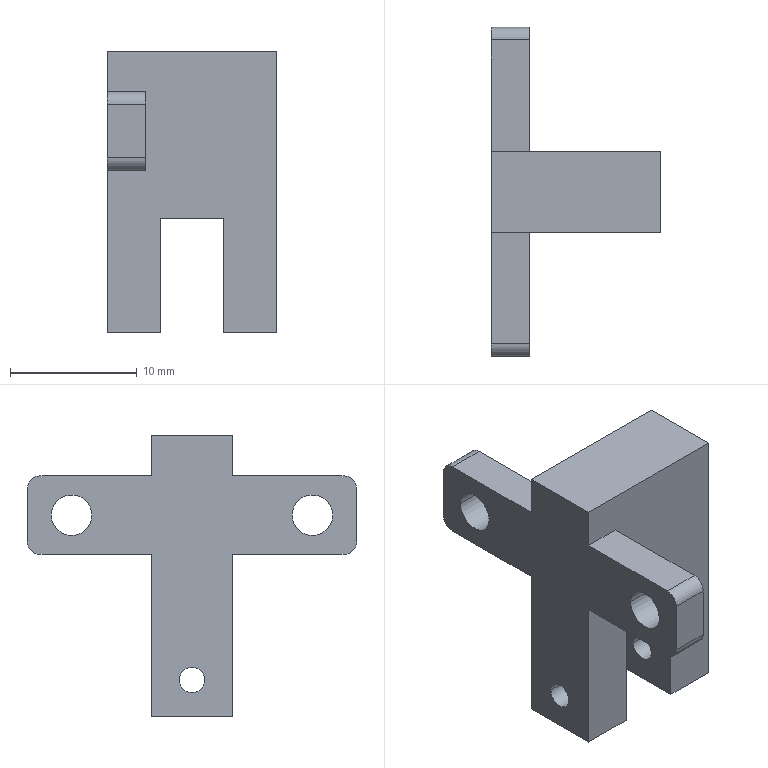Component | SolidWorks | V1ZHXTRR60SecondarySB1-1_v1ZHXTEE-SX672SB1-1 | 1 solid | 30 faces | box 13.4 x 26 x 22.2 mm | volume 1903 mm3 | plane 18 | cylinder 12 | commonest cylinder face diameters 2 x8 3.2 x4
STEP:
#1=COLOUR_RGB('',0.7922,0.8196,0.9333);
#2=FILL_AREA_STYLE_COLOUR('',#1);
#3=FILL_AREA_STYLE('',(#2));
#4=SURFACE_STYLE_FILL_AREA(#3);
#5=SURFACE_SIDE_STYLE('',(#4));
#6=SURFACE_STYLE_USAGE(.BOTH.,#5);
#7=PRESENTATION_STYLE_ASSIGNMENT((#6));
#8=CARTESIAN_POINT('',(9.509,-8.474,18.97));
#9=VERTEX_POINT('',#8);
#10=CARTESIAN_POINT('',(9.509,-8.348,18.97));
#11=VERTEX_POINT('',#10);
#12=CARTESIAN_POINT('',(9.509,-8.411,18.97));
#13=DIRECTION('',(-1.,-0.,-0.));
#14=DIRECTION('',(0.,-1.,-0.));
#15=AXIS2_PLACEMENT_3D('',#12,#13,#14);
#16=CIRCLE('',#15,0.06299);
#17=EDGE_CURVE('',#9,#11,#16,.T.);
#18=ORIENTED_EDGE('',*,*,#17,.T.);
#19=CARTESIAN_POINT('',(9.627,-8.348,18.97));
#20=VERTEX_POINT('',#19);
#21=CARTESIAN_POINT('',(9.627,-8.348,18.97));
#22=DIRECTION('',(1.,0.,0.));
#23=VECTOR('',#22,39.37);
#24=LINE('',#21,#23);
#25=EDGE_CURVE('',#11,#20,#24,.T.);
#26=ORIENTED_EDGE('',*,*,#25,.T.);
#27=CARTESIAN_POINT('',(9.627,-8.474,18.97));
#28=VERTEX_POINT('',#27);
#29=CARTESIAN_POINT('',(9.627,-8.411,18.97));
#30=DIRECTION('',(-1.,-0.,-0.));
#31=DIRECTION('',(0.,-1.,-0.));
#32=AXIS2_PLACEMENT_3D('',#29,#30,#31);
#33=CIRCLE('',#32,0.06299);
#34=EDGE_CURVE('',#28,#20,#33,.T.);
#35=ORIENTED_EDGE('',*,*,#34,.F.);
#36=CARTESIAN_POINT('',(9.627,-8.474,18.97));
#37=DIRECTION('',(1.,0.,0.));
#38=VECTOR('',#37,39.37);
#39=LINE('',#36,#38);
#40=EDGE_CURVE('',#9,#28,#39,.T.);
#41=ORIENTED_EDGE('',*,*,#40,.F.);
#42=EDGE_LOOP('',(#18,#26,#35,#41));
#43=FACE_OUTER_BOUND('',#42,.T.);
#44=CARTESIAN_POINT('',(9.627,-8.411,18.97));
#45=DIRECTION('',(1.,0.,0.));
#46=DIRECTION('',(0.,-1.,-0.));
#47=AXIS2_PLACEMENT_3D('',#44,#45,#46);
#48=CYLINDRICAL_SURFACE('',#47,0.06299);
#49=ADVANCED_FACE('',(#43),#48,.F.);
#50=CARTESIAN_POINT('',(9.509,-7.726,18.97));
#51=VERTEX_POINT('',#50);
#52=CARTESIAN_POINT('',(9.509,-7.6,18.97));
#53=VERTEX_POINT('',#52);
#54=CARTESIAN_POINT('',(9.509,-7.663,18.97));
#55=DIRECTION('',(-1.,-0.,-0.));
#56=DIRECTION('',(0.,-1.,-0.));
#57=AXIS2_PLACEMENT_3D('',#54,#55,#56);
#58=CIRCLE('',#57,0.06299);
#59=EDGE_CURVE('',#51,#53,#58,.T.);
#60=ORIENTED_EDGE('',*,*,#59,.T.);
#61=CARTESIAN_POINT('',(9.627,-7.6,18.97));
#62=VERTEX_POINT('',#61);
#63=CARTESIAN_POINT('',(9.627,-7.6,18.97));
#64=DIRECTION('',(1.,0.,0.));
#65=VECTOR('',#64,39.37);
#66=LINE('',#63,#65);
#67=EDGE_CURVE('',#53,#62,#66,.T.);
#68=ORIENTED_EDGE('',*,*,#67,.T.);
#69=CARTESIAN_POINT('',(9.627,-7.726,18.97));
#70=VERTEX_POINT('',#69);
#71=CARTESIAN_POINT('',(9.627,-7.663,18.97));
#72=DIRECTION('',(-1.,-0.,-0.));
#73=DIRECTION('',(0.,-1.,-0.));
#74=AXIS2_PLACEMENT_3D('',#71,#72,#73);
#75=CIRCLE('',#74,0.06299);
#76=EDGE_CURVE('',#70,#62,#75,.T.);
#77=ORIENTED_EDGE('',*,*,#76,.F.);
#78=CARTESIAN_POINT('',(9.627,-7.726,18.97));
#79=DIRECTION('',(1.,0.,0.));
#80=VECTOR('',#79,39.37);
#81=LINE('',#78,#80);
#82=EDGE_CURVE('',#51,#70,#81,.T.);
#83=ORIENTED_EDGE('',*,*,#82,.F.);
#84=EDGE_LOOP('',(#60,#68,#77,#83));
#85=FACE_OUTER_BOUND('',#84,.T.);
#86=CARTESIAN_POINT('',(9.627,-7.663,18.97));
#87=DIRECTION('',(1.,0.,0.));
#88=DIRECTION('',(0.,-1.,-0.));
#89=AXIS2_PLACEMENT_3D('',#86,#87,#88);
#90=CYLINDRICAL_SURFACE('',#89,0.06299);
#91=ADVANCED_FACE('',(#85),#90,.F.);
#92=CARTESIAN_POINT('',(9.509,-8.076,18.458));
#93=VERTEX_POINT('',#92);
#94=CARTESIAN_POINT('',(9.509,-7.997,18.458));
#95=VERTEX_POINT('',#94);
#96=CARTESIAN_POINT('',(9.509,-8.037,18.458));
#97=DIRECTION('',(-1.,-0.,-0.));
#98=DIRECTION('',(0.,-1.,-0.));
#99=AXIS2_PLACEMENT_3D('',#96,#97,#98);
#100=CIRCLE('',#99,0.03937);
#101=EDGE_CURVE('',#93,#95,#100,.T.);
#102=ORIENTED_EDGE('',*,*,#101,.T.);
#103=CARTESIAN_POINT('',(9.674,-7.997,18.458));
#104=VERTEX_POINT('',#103);
#105=CARTESIAN_POINT('',(10.036,-7.997,18.458));
#106=DIRECTION('',(1.,0.,0.));
#107=VECTOR('',#106,39.37);
#108=LINE('',#105,#107);
#109=EDGE_CURVE('',#95,#104,#108,.T.);
#110=ORIENTED_EDGE('',*,*,#109,.T.);
#111=CARTESIAN_POINT('',(9.674,-8.076,18.458));
#112=VERTEX_POINT('',#111);
#113=CARTESIAN_POINT('',(9.674,-8.037,18.458));
#114=DIRECTION('',(-1.,-0.,-0.));
#115=DIRECTION('',(0.,-1.,-0.));
#116=AXIS2_PLACEMENT_3D('',#113,#114,#115);
#117=CIRCLE('',#116,0.03937);
#118=EDGE_CURVE('',#112,#104,#117,.T.);
#119=ORIENTED_EDGE('',*,*,#118,.F.);
#120=CARTESIAN_POINT('',(10.036,-8.076,18.458));
#121=DIRECTION('',(1.,0.,0.));
#122=VECTOR('',#121,39.37);
#123=LINE('',#120,#122);
#124=EDGE_CURVE('',#93,#112,#123,.T.);
#125=ORIENTED_EDGE('',*,*,#124,.F.);
#126=EDGE_LOOP('',(#102,#110,#119,#125));
#127=FACE_OUTER_BOUND('',#126,.T.);
#128=CARTESIAN_POINT('',(10.036,-8.037,18.458));
#129=DIRECTION('',(1.,0.,0.));
#130=DIRECTION('',(0.,-1.,-0.));
#131=AXIS2_PLACEMENT_3D('',#128,#129,#130);
#132=CYLINDRICAL_SURFACE('',#131,0.03937);
#133=ADVANCED_FACE('',(#127),#132,.F.);
#134=CARTESIAN_POINT('',(9.871,-8.076,18.458));
#135=VERTEX_POINT('',#134);
#136=CARTESIAN_POINT('',(9.871,-7.997,18.458));
#137=VERTEX_POINT('',#136);
#138=CARTESIAN_POINT('',(9.871,-8.037,18.458));
#139=DIRECTION('',(-1.,-0.,-0.));
#140=DIRECTION('',(0.,-1.,-0.));
#141=AXIS2_PLACEMENT_3D('',#138,#139,#140);
#142=CIRCLE('',#141,0.03937);
#143=EDGE_CURVE('',#135,#137,#142,.T.);
#144=ORIENTED_EDGE('',*,*,#143,.T.);
#145=CARTESIAN_POINT('',(10.036,-7.997,18.458));
#146=VERTEX_POINT('',#145);
#147=CARTESIAN_POINT('',(10.036,-7.997,18.458));
#148=DIRECTION('',(1.,0.,0.));
#149=VECTOR('',#148,39.37);
#150=LINE('',#147,#149);
#151=EDGE_CURVE('',#137,#146,#150,.T.);
#152=ORIENTED_EDGE('',*,*,#151,.T.);
#153=CARTESIAN_POINT('',(10.036,-8.076,18.458));
#154=VERTEX_POINT('',#153);
#155=CARTESIAN_POINT('',(10.036,-8.037,18.458));
#156=DIRECTION('',(1.,0.,0.));
#157=DIRECTION('',(0.,-1.,-0.));
#158=AXIS2_PLACEMENT_3D('',#155,#156,#157);
#159=CIRCLE('',#158,0.03937);
#160=EDGE_CURVE('',#146,#154,#159,.T.);
#161=ORIENTED_EDGE('',*,*,#160,.T.);
#162=CARTESIAN_POINT('',(10.036,-8.076,18.458));
#163=DIRECTION('',(1.,0.,0.));
#164=VECTOR('',#163,39.37);
#165=LINE('',#162,#164);
#166=EDGE_CURVE('',#135,#154,#165,.T.);
#167=ORIENTED_EDGE('',*,*,#166,.F.);
#168=EDGE_LOOP('',(#144,#152,#161,#167));
#169=FACE_OUTER_BOUND('',#168,.T.);
#170=CARTESIAN_POINT('',(10.036,-8.037,18.458));
#171=DIRECTION('',(1.,0.,0.));
#172=DIRECTION('',(0.,-1.,-0.));
#173=AXIS2_PLACEMENT_3D('',#170,#171,#172);
#174=CYLINDRICAL_SURFACE('',#173,0.03937);
#175=ADVANCED_FACE('',(#169),#174,.F.);
#176=CARTESIAN_POINT('',(9.509,-7.525,19.053));
#177=VERTEX_POINT('',#176);
#178=CARTESIAN_POINT('',(9.509,-7.564,19.092));
#179=VERTEX_POINT('',#178);
#180=CARTESIAN_POINT('',(9.509,-7.564,19.053));
#181=DIRECTION('',(1.,0.,0.));
#182=DIRECTION('',(-0.,1.,0.));
#183=AXIS2_PLACEMENT_3D('',#180,#181,#182);
#184=CIRCLE('',#183,0.03937);
#185=EDGE_CURVE('',#177,#179,#184,.T.);
#186=ORIENTED_EDGE('',*,*,#185,.F.);
#187=CARTESIAN_POINT('',(9.509,-7.525,18.887));
#188=VERTEX_POINT('',#187);
#189=CARTESIAN_POINT('',(9.509,-7.525,19.218));
#190=DIRECTION('',(-0.,-0.,1.));
#191=VECTOR('',#190,39.37);
#192=LINE('',#189,#191);
#193=EDGE_CURVE('',#188,#177,#192,.T.);
#194=ORIENTED_EDGE('',*,*,#193,.F.);
#195=CARTESIAN_POINT('',(9.509,-7.564,18.848));
#196=VERTEX_POINT('',#195);
#197=CARTESIAN_POINT('',(9.509,-7.564,18.887));
#198=DIRECTION('',(1.,0.,0.));
#199=DIRECTION('',(-0.,1.,0.));
#200=AXIS2_PLACEMENT_3D('',#197,#198,#199);
#201=CIRCLE('',#200,0.03937);
#202=EDGE_CURVE('',#196,#188,#201,.T.);
#203=ORIENTED_EDGE('',*,*,#202,.F.);
#204=CARTESIAN_POINT('',(9.509,-7.911,18.848));
#205=VERTEX_POINT('',#204);
#206=CARTESIAN_POINT('',(9.509,-7.911,18.848));
#207=DIRECTION('',(-0.,1.,0.));
#208=VECTOR('',#207,39.37);
#209=LINE('',#206,#208);
#210=EDGE_CURVE('',#205,#196,#209,.T.);
#211=ORIENTED_EDGE('',*,*,#210,.F.);
#212=CARTESIAN_POINT('',(9.509,-7.911,18.344));
#213=VERTEX_POINT('',#212);
#214=CARTESIAN_POINT('',(9.509,-7.911,19.218));
#215=DIRECTION('',(-0.,-0.,1.));
#216=VECTOR('',#215,39.37);
#217=LINE('',#214,#216);
#218=EDGE_CURVE('',#213,#205,#217,.T.);
#219=ORIENTED_EDGE('',*,*,#218,.F.);
#220=CARTESIAN_POINT('',(9.509,-8.163,18.344));
#221=VERTEX_POINT('',#220);
#222=CARTESIAN_POINT('',(9.509,-7.911,18.344));
#223=DIRECTION('',(-0.,1.,0.));
#224=VECTOR('',#223,39.37);
#225=LINE('',#222,#224);
#226=EDGE_CURVE('',#221,#213,#225,.T.);
#227=ORIENTED_EDGE('',*,*,#226,.F.);
#228=CARTESIAN_POINT('',(9.509,-8.163,18.848));
#229=VERTEX_POINT('',#228);
#230=CARTESIAN_POINT('',(9.509,-8.163,19.218));
#231=DIRECTION('',(0.,0.,-1.));
#232=VECTOR('',#231,39.37);
#233=LINE('',#230,#232);
#234=EDGE_CURVE('',#229,#221,#233,.T.);
#235=ORIENTED_EDGE('',*,*,#234,.F.);
#236=CARTESIAN_POINT('',(9.509,-8.509,18.848));
#237=VERTEX_POINT('',#236);
#238=CARTESIAN_POINT('',(9.509,-7.911,18.848));
#239=DIRECTION('',(-0.,1.,0.));
#240=VECTOR('',#239,39.37);
#241=LINE('',#238,#240);
#242=EDGE_CURVE('',#237,#229,#241,.T.);
#243=ORIENTED_EDGE('',*,*,#242,.F.);
#244=CARTESIAN_POINT('',(9.509,-8.548,18.887));
#245=VERTEX_POINT('',#244);
#246=CARTESIAN_POINT('',(9.509,-8.509,18.887));
#247=DIRECTION('',(1.,0.,0.));
#248=DIRECTION('',(-0.,1.,0.));
#249=AXIS2_PLACEMENT_3D('',#246,#247,#248);
#250=CIRCLE('',#249,0.03937);
#251=EDGE_CURVE('',#245,#237,#250,.T.);
#252=ORIENTED_EDGE('',*,*,#251,.F.);
#253=CARTESIAN_POINT('',(9.509,-8.548,19.053));
#254=VERTEX_POINT('',#253);
#255=CARTESIAN_POINT('',(9.509,-8.548,19.218));
#256=DIRECTION('',(0.,0.,-1.));
#257=VECTOR('',#256,39.37);
#258=LINE('',#255,#257);
#259=EDGE_CURVE('',#254,#245,#258,.T.);
#260=ORIENTED_EDGE('',*,*,#259,.F.);
#261=CARTESIAN_POINT('',(9.509,-8.509,19.092));
#262=VERTEX_POINT('',#261);
#263=CARTESIAN_POINT('',(9.509,-8.509,19.053));
#264=DIRECTION('',(1.,0.,0.));
#265=DIRECTION('',(-0.,1.,0.));
#266=AXIS2_PLACEMENT_3D('',#263,#264,#265);
#267=CIRCLE('',#266,0.03937);
#268=EDGE_CURVE('',#262,#254,#267,.T.);
#269=ORIENTED_EDGE('',*,*,#268,.F.);
#270=CARTESIAN_POINT('',(9.509,-8.163,19.092));
#271=VERTEX_POINT('',#270);
#272=CARTESIAN_POINT('',(9.509,-7.911,19.092));
#273=DIRECTION('',(0.,-1.,-0.));
#274=VECTOR('',#273,39.37);
#275=LINE('',#272,#274);
#276=EDGE_CURVE('',#271,#262,#275,.T.);
#277=ORIENTED_EDGE('',*,*,#276,.F.);
#278=CARTESIAN_POINT('',(9.509,-8.163,19.218));
#279=VERTEX_POINT('',#278);
#280=CARTESIAN_POINT('',(9.509,-8.163,19.218));
#281=DIRECTION('',(0.,0.,-1.));
#282=VECTOR('',#281,39.37);
#283=LINE('',#280,#282);
#284=EDGE_CURVE('',#279,#271,#283,.T.);
#285=ORIENTED_EDGE('',*,*,#284,.F.);
#286=CARTESIAN_POINT('',(9.509,-7.911,19.218));
#287=VERTEX_POINT('',#286);
#288=CARTESIAN_POINT('',(9.509,-7.911,19.218));
#289=DIRECTION('',(0.,-1.,-0.));
#290=VECTOR('',#289,39.37);
#291=LINE('',#288,#290);
#292=EDGE_CURVE('',#287,#279,#291,.T.);
#293=ORIENTED_EDGE('',*,*,#292,.F.);
#294=CARTESIAN_POINT('',(9.509,-7.911,19.092));
#295=VERTEX_POINT('',#294);
#296=CARTESIAN_POINT('',(9.509,-7.911,19.218));
#297=DIRECTION('',(-0.,-0.,1.));
#298=VECTOR('',#297,39.37);
#299=LINE('',#296,#298);
#300=EDGE_CURVE('',#295,#287,#299,.T.);
#301=ORIENTED_EDGE('',*,*,#300,.F.);
#302=CARTESIAN_POINT('',(9.509,-7.911,19.092));
#303=DIRECTION('',(0.,-1.,-0.));
#304=VECTOR('',#303,39.37);
#305=LINE('',#302,#304);
#306=EDGE_CURVE('',#179,#295,#305,.T.);
#307=ORIENTED_EDGE('',*,*,#306,.F.);
#308=EDGE_LOOP('',(#186,#194,#203,#211,#219,#227,#235,#243,#252,#260,#269,#277,#285,#293,#301,#307));
#309=FACE_OUTER_BOUND('',#308,.T.);
#310=ORIENTED_EDGE('',*,*,#17,.F.);
#311=CARTESIAN_POINT('',(9.509,-8.411,18.97));
#312=DIRECTION('',(-1.,-0.,-0.));
#313=DIRECTION('',(0.,-1.,-0.));
#314=AXIS2_PLACEMENT_3D('',#311,#312,#313);
#315=CIRCLE('',#314,0.06299);
#316=EDGE_CURVE('',#11,#9,#315,.T.);
#317=ORIENTED_EDGE('',*,*,#316,.F.);
#318=EDGE_LOOP('',(#310,#317));
#319=FACE_BOUND('',#318,.T.);
#320=ORIENTED_EDGE('',*,*,#59,.F.);
#321=CARTESIAN_POINT('',(9.509,-7.663,18.97));
#322=DIRECTION('',(-1.,-0.,-0.));
#323=DIRECTION('',(0.,-1.,-0.));
#324=AXIS2_PLACEMENT_3D('',#321,#322,#323);
#325=CIRCLE('',#324,0.06299);
#326=EDGE_CURVE('',#53,#51,#325,.T.);
#327=ORIENTED_EDGE('',*,*,#326,.F.);
#328=EDGE_LOOP('',(#320,#327));
#329=FACE_BOUND('',#328,.T.);
#330=ORIENTED_EDGE('',*,*,#101,.F.);
#331=CARTESIAN_POINT('',(9.509,-8.037,18.458));
#332=DIRECTION('',(-1.,-0.,-0.));
#333=DIRECTION('',(0.,-1.,-0.));
#334=AXIS2_PLACEMENT_3D('',#331,#332,#333);
#335=CIRCLE('',#334,0.03937);
#336=EDGE_CURVE('',#95,#93,#335,.T.);
#337=ORIENTED_EDGE('',*,*,#336,.F.);
#338=EDGE_LOOP('',(#330,#337));
#339=FACE_BOUND('',#338,.T.);
#340=CARTESIAN_POINT('',(9.509,-7.911,19.218));
#341=DIRECTION('',(1.,0.,0.));
#342=DIRECTION('',(0.,-1.,-0.));
#343=AXIS2_PLACEMENT_3D('',#340,#341,#342);
#344=PLANE('',#343);
#345=ADVANCED_FACE('',(#309,#319,#329,#339),#344,.F.);
#346=ORIENTED_EDGE('',*,*,#306,.T.);
#347=CARTESIAN_POINT('',(9.627,-7.911,19.092));
#348=VERTEX_POINT('',#347);
#349=CARTESIAN_POINT('',(9.627,-7.911,19.092));
#350=DIRECTION('',(1.,0.,0.));
#351=VECTOR('',#350,39.37);
#352=LINE('',#349,#351);
#353=EDGE_CURVE('',#295,#348,#352,.T.);
#354=ORIENTED_EDGE('',*,*,#353,.T.);
#355=CARTESIAN_POINT('',(9.627,-7.564,19.092));
#356=VERTEX_POINT('',#355);
#357=CARTESIAN_POINT('',(9.627,-7.911,19.092));
#358=DIRECTION('',(-0.,1.,0.));
#359=VECTOR('',#358,39.37);
#360=LINE('',#357,#359);
#361=EDGE_CURVE('',#348,#356,#360,.T.);
#362=ORIENTED_EDGE('',*,*,#361,.T.);
#363=CARTESIAN_POINT('',(9.627,-7.564,19.092));
#364=DIRECTION('',(-1.,-0.,-0.));
#365=VECTOR('',#364,39.37);
#366=LINE('',#363,#365);
#367=EDGE_CURVE('',#356,#179,#366,.T.);
#368=ORIENTED_EDGE('',*,*,#367,.T.);
#369=EDGE_LOOP('',(#346,#354,#362,#368));
#370=FACE_OUTER_BOUND('',#369,.T.);
#371=CARTESIAN_POINT('',(9.627,-7.911,19.092));
#372=DIRECTION('',(-0.,-0.,1.));
#373=DIRECTION('',(0.,-1.,-0.));
#374=AXIS2_PLACEMENT_3D('',#371,#372,#373);
#375=PLANE('',#374);
#376=ADVANCED_FACE('',(#370),#375,.T.);
#377=CARTESIAN_POINT('',(9.627,-7.525,19.053));
#378=VERTEX_POINT('',#377);
#379=CARTESIAN_POINT('',(9.627,-7.525,18.887));
#380=VERTEX_POINT('',#379);
#381=CARTESIAN_POINT('',(9.627,-7.525,18.848));
#382=DIRECTION('',(0.,0.,-1.));
#383=VECTOR('',#382,39.37);
#384=LINE('',#381,#383);
#385=EDGE_CURVE('',#378,#380,#384,.T.);
#386=ORIENTED_EDGE('',*,*,#385,.T.);
#387=CARTESIAN_POINT('',(9.627,-7.525,18.887));
#388=DIRECTION('',(-1.,-0.,-0.));
#389=VECTOR('',#388,39.37);
#390=LINE('',#387,#389);
#391=EDGE_CURVE('',#380,#188,#390,.T.);
#392=ORIENTED_EDGE('',*,*,#391,.T.);
#393=ORIENTED_EDGE('',*,*,#193,.T.);
#394=CARTESIAN_POINT('',(9.627,-7.525,19.053));
#395=DIRECTION('',(1.,0.,0.));
#396=VECTOR('',#395,39.37);
#397=LINE('',#394,#396);
#398=EDGE_CURVE('',#177,#378,#397,.T.);
#399=ORIENTED_EDGE('',*,*,#398,.T.);
#400=EDGE_LOOP('',(#386,#392,#393,#399));
#401=FACE_OUTER_BOUND('',#400,.T.);
#402=CARTESIAN_POINT('',(9.627,-7.525,18.848));
#403=DIRECTION('',(-0.,1.,0.));
#404=DIRECTION('',(1.,0.,0.));
#405=AXIS2_PLACEMENT_3D('',#402,#403,#404);
#406=PLANE('',#405);
#407=ADVANCED_FACE('',(#401),#406,.T.);
#408=CARTESIAN_POINT('',(9.627,-7.564,18.848));
#409=VERTEX_POINT('',#408);
#410=CARTESIAN_POINT('',(9.627,-7.911,18.848));
#411=VERTEX_POINT('',#410);
#412=CARTESIAN_POINT('',(9.627,-7.911,18.848));
#413=DIRECTION('',(0.,-1.,-0.));
#414=VECTOR('',#413,39.37);
#415=LINE('',#412,#414);
#416=EDGE_CURVE('',#409,#411,#415,.T.);
#417=ORIENTED_EDGE('',*,*,#416,.T.);
#418=CARTESIAN_POINT('',(9.627,-7.911,18.848));
#419=DIRECTION('',(-1.,-0.,-0.));
#420=VECTOR('',#419,39.37);
#421=LINE('',#418,#420);
#422=EDGE_CURVE('',#411,#205,#421,.T.);
#423=ORIENTED_EDGE('',*,*,#422,.T.);
#424=ORIENTED_EDGE('',*,*,#210,.T.);
#425=CARTESIAN_POINT('',(9.627,-7.564,18.848));
#426=DIRECTION('',(1.,0.,0.));
#427=VECTOR('',#426,39.37);
#428=LINE('',#425,#427);
#429=EDGE_CURVE('',#196,#409,#428,.T.);
#430=ORIENTED_EDGE('',*,*,#429,.T.);
#431=EDGE_LOOP('',(#417,#423,#424,#430));
#432=FACE_OUTER_BOUND('',#431,.T.);
#433=CARTESIAN_POINT('',(9.627,-7.911,18.848));
#434=DIRECTION('',(0.,0.,-1.));
#435=DIRECTION('',(-0.,1.,0.));
#436=AXIS2_PLACEMENT_3D('',#433,#434,#435);
#437=PLANE('',#436);
#438=ADVANCED_FACE('',(#432),#437,.T.);
#439=CARTESIAN_POINT('',(9.627,-7.911,18.344));
#440=DIRECTION('',(0.,0.,-1.));
#441=VECTOR('',#440,39.37);
#442=LINE('',#439,#441);
#443=EDGE_CURVE('',#348,#411,#442,.T.);
#444=ORIENTED_EDGE('',*,*,#443,.F.);
#445=ORIENTED_EDGE('',*,*,#353,.F.);
#446=ORIENTED_EDGE('',*,*,#300,.T.);
#447=CARTESIAN_POINT('',(10.036,-7.911,19.218));
#448=VERTEX_POINT('',#447);
#449=CARTESIAN_POINT('',(9.509,-7.911,19.218));
#450=DIRECTION('',(-1.,-0.,-0.));
#451=VECTOR('',#450,39.37);
#452=LINE('',#449,#451);
#453=EDGE_CURVE('',#448,#287,#452,.T.);
#454=ORIENTED_EDGE('',*,*,#453,.F.);
#455=CARTESIAN_POINT('',(10.036,-7.911,18.344));
#456=VERTEX_POINT('',#455);
#457=CARTESIAN_POINT('',(10.036,-7.911,18.344));
#458=DIRECTION('',(-0.,-0.,1.));
#459=VECTOR('',#458,39.37);
#460=LINE('',#457,#459);
#461=EDGE_CURVE('',#456,#448,#460,.T.);
#462=ORIENTED_EDGE('',*,*,#461,.F.);
#463=CARTESIAN_POINT('',(9.871,-7.911,18.344));
#464=VERTEX_POINT('',#463);
#465=CARTESIAN_POINT('',(9.509,-7.911,18.344));
#466=DIRECTION('',(1.,0.,0.));
#467=VECTOR('',#466,39.37);
#468=LINE('',#465,#467);
#469=EDGE_CURVE('',#464,#456,#468,.T.);
#470=ORIENTED_EDGE('',*,*,#469,.F.);
#471=CARTESIAN_POINT('',(9.871,-7.911,18.698));
#472=VERTEX_POINT('',#471);
#473=CARTESIAN_POINT('',(9.871,-7.911,18.344));
#474=DIRECTION('',(0.,0.,-1.));
#475=VECTOR('',#474,39.37);
#476=LINE('',#473,#475);
#477=EDGE_CURVE('',#472,#464,#476,.T.);
#478=ORIENTED_EDGE('',*,*,#477,.F.);
#479=CARTESIAN_POINT('',(9.674,-7.911,18.698));
#480=VERTEX_POINT('',#479);
#481=CARTESIAN_POINT('',(9.509,-7.911,18.698));
#482=DIRECTION('',(1.,0.,0.));
#483=VECTOR('',#482,39.37);
#484=LINE('',#481,#483);
#485=EDGE_CURVE('',#480,#472,#484,.T.);
#486=ORIENTED_EDGE('',*,*,#485,.F.);
#487=CARTESIAN_POINT('',(9.674,-7.911,18.344));
#488=VERTEX_POINT('',#487);
#489=CARTESIAN_POINT('',(9.674,-7.911,18.344));
#490=DIRECTION('',(-0.,-0.,1.));
#491=VECTOR('',#490,39.37);
#492=LINE('',#489,#491);
#493=EDGE_CURVE('',#488,#480,#492,.T.);
#494=ORIENTED_EDGE('',*,*,#493,.F.);
#495=CARTESIAN_POINT('',(9.509,-7.911,18.344));
#496=DIRECTION('',(1.,0.,0.));
#497=VECTOR('',#496,39.37);
#498=LINE('',#495,#497);
#499=EDGE_CURVE('',#213,#488,#498,.T.);
#500=ORIENTED_EDGE('',*,*,#499,.F.);
#501=ORIENTED_EDGE('',*,*,#218,.T.);
#502=ORIENTED_EDGE('',*,*,#422,.F.);
#503=EDGE_LOOP('',(#444,#445,#446,#454,#462,#470,#478,#486,#494,#500,#501,#502));
#504=FACE_OUTER_BOUND('',#503,.T.);
#505=CARTESIAN_POINT('',(9.509,-7.911,18.344));
#506=DIRECTION('',(0.,-1.,-0.));
#507=DIRECTION('',(-1.,-0.,-0.));
#508=AXIS2_PLACEMENT_3D('',#505,#506,#507);
#509=PLANE('',#508);
#510=ADVANCED_FACE('',(#504),#509,.F.);
#511=CARTESIAN_POINT('',(9.674,-8.163,18.344));
#512=VERTEX_POINT('',#511);
#513=CARTESIAN_POINT('',(9.674,-7.911,18.344));
#514=DIRECTION('',(-0.,1.,0.));
#515=VECTOR('',#514,39.37);
#516=LINE('',#513,#515);
#517=EDGE_CURVE('',#512,#488,#516,.T.);
#518=ORIENTED_EDGE('',*,*,#517,.F.);
#519=CARTESIAN_POINT('',(9.509,-8.163,18.344));
#520=DIRECTION('',(1.,0.,-0.));
#521=VECTOR('',#520,39.37);
#522=LINE('',#519,#521);
#523=EDGE_CURVE('',#221,#512,#522,.T.);
#524=ORIENTED_EDGE('',*,*,#523,.F.);
#525=ORIENTED_EDGE('',*,*,#226,.T.);
#526=ORIENTED_EDGE('',*,*,#499,.T.);
#527=EDGE_LOOP('',(#518,#524,#525,#526));
#528=FACE_OUTER_BOUND('',#527,.T.);
#529=CARTESIAN_POINT('',(9.509,-7.911,18.344));
#530=DIRECTION('',(0.,-0.,1.));
#531=DIRECTION('',(1.,0.,-0.));
#532=AXIS2_PLACEMENT_3D('',#529,#530,#531);
#533=PLANE('',#532);
#534=ADVANCED_FACE('',(#528),#533,.F.);
#535=CARTESIAN_POINT('',(10.036,-8.163,19.218));
#536=VERTEX_POINT('',#535);
#537=CARTESIAN_POINT('',(9.509,-8.163,19.218));
#538=DIRECTION('',(-1.,-0.,-0.));
#539=VECTOR('',#538,39.37);
#540=LINE('',#537,#539);
#541=EDGE_CURVE('',#536,#279,#540,.T.);
#542=ORIENTED_EDGE('',*,*,#541,.T.);
#543=ORIENTED_EDGE('',*,*,#284,.T.);
#544=CARTESIAN_POINT('',(9.627,-8.163,19.092));
#545=VERTEX_POINT('',#544);
#546=CARTESIAN_POINT('',(9.509,-8.163,19.092));
#547=DIRECTION('',(1.,0.,0.));
#548=VECTOR('',#547,39.37);
#549=LINE('',#546,#548);
#550=EDGE_CURVE('',#271,#545,#549,.T.);
#551=ORIENTED_EDGE('',*,*,#550,.T.);
#552=CARTESIAN_POINT('',(9.627,-8.163,18.848));
#553=VERTEX_POINT('',#552);
#554=CARTESIAN_POINT('',(9.627,-8.163,18.344));
#555=DIRECTION('',(0.,0.,-1.));
#556=VECTOR('',#555,39.37);
#557=LINE('',#554,#556);
#558=EDGE_CURVE('',#545,#553,#557,.T.);
#559=ORIENTED_EDGE('',*,*,#558,.T.);
#560=CARTESIAN_POINT('',(9.509,-8.163,18.848));
#561=DIRECTION('',(-1.,-0.,-0.));
#562=VECTOR('',#561,39.37);
#563=LINE('',#560,#562);
#564=EDGE_CURVE('',#553,#229,#563,.T.);
#565=ORIENTED_EDGE('',*,*,#564,.T.);
#566=ORIENTED_EDGE('',*,*,#234,.T.);
#567=ORIENTED_EDGE('',*,*,#523,.T.);
#568=CARTESIAN_POINT('',(9.674,-8.163,18.698));
#569=VERTEX_POINT('',#568);
#570=CARTESIAN_POINT('',(9.674,-8.163,18.344));
#571=DIRECTION('',(-0.,-0.,1.));
#572=VECTOR('',#571,39.37);
#573=LINE('',#570,#572);
#574=EDGE_CURVE('',#512,#569,#573,.T.);
#575=ORIENTED_EDGE('',*,*,#574,.T.);
#576=CARTESIAN_POINT('',(9.871,-8.163,18.698));
#577=VERTEX_POINT('',#576);
#578=CARTESIAN_POINT('',(9.509,-8.163,18.698));
#579=DIRECTION('',(1.,0.,0.));
#580=VECTOR('',#579,39.37);
#581=LINE('',#578,#580);
#582=EDGE_CURVE('',#569,#577,#581,.T.);
#583=ORIENTED_EDGE('',*,*,#582,.T.);
#584=CARTESIAN_POINT('',(9.871,-8.163,18.344));
#585=VERTEX_POINT('',#584);
#586=CARTESIAN_POINT('',(9.871,-8.163,18.344));
#587=DIRECTION('',(0.,0.,-1.));
#588=VECTOR('',#587,39.37);
#589=LINE('',#586,#588);
#590=EDGE_CURVE('',#577,#585,#589,.T.);
#591=ORIENTED_EDGE('',*,*,#590,.T.);
#592=CARTESIAN_POINT('',(10.036,-8.163,18.344));
#593=VERTEX_POINT('',#592);
#594=CARTESIAN_POINT('',(9.509,-8.163,18.344));
#595=DIRECTION('',(1.,0.,0.));
#596=VECTOR('',#595,39.37);
#597=LINE('',#594,#596);
#598=EDGE_CURVE('',#585,#593,#597,.T.);
#599=ORIENTED_EDGE('',*,*,#598,.T.);
#600=CARTESIAN_POINT('',(10.036,-8.163,18.344));
#601=DIRECTION('',(-0.,-0.,1.));
#602=VECTOR('',#601,39.37);
#603=LINE('',#600,#602);
#604=EDGE_CURVE('',#593,#536,#603,.T.);
#605=ORIENTED_EDGE('',*,*,#604,.T.);
#606=EDGE_LOOP('',(#542,#543,#551,#559,#565,#566,#567,#575,#583,#591,#599,#605));
#607=FACE_OUTER_BOUND('',#606,.T.);
#608=CARTESIAN_POINT('',(9.509,-8.163,18.344));
#609=DIRECTION('',(0.,-1.,-0.));
#610=DIRECTION('',(-1.,-0.,-0.));
#611=AXIS2_PLACEMENT_3D('',#608,#609,#610);
#612=PLANE('',#611);
#613=ADVANCED_FACE('',(#607),#612,.T.);
#614=ORIENTED_EDGE('',*,*,#242,.T.);
#615=ORIENTED_EDGE('',*,*,#564,.F.);
#616=CARTESIAN_POINT('',(9.627,-8.509,18.848));
#617=VERTEX_POINT('',#616);
#618=CARTESIAN_POINT('',(9.627,-8.163,18.848));
#619=DIRECTION('',(0.,-1.,-0.));
#620=VECTOR('',#619,39.37);
#621=LINE('',#618,#620);
#622=EDGE_CURVE('',#553,#617,#621,.T.);
#623=ORIENTED_EDGE('',*,*,#622,.T.);
#624=CARTESIAN_POINT('',(9.627,-8.509,18.848));
#625=DIRECTION('',(-1.,-0.,-0.));
#626=VECTOR('',#625,39.37);
#627=LINE('',#624,#626);
#628=EDGE_CURVE('',#617,#237,#627,.T.);
#629=ORIENTED_EDGE('',*,*,#628,.T.);
#630=EDGE_LOOP('',(#614,#615,#623,#629));
#631=FACE_OUTER_BOUND('',#630,.T.);
#632=CARTESIAN_POINT('',(9.627,-8.163,18.848));
#633=DIRECTION('',(0.,0.,-1.));
#634=DIRECTION('',(-0.,1.,0.));
#635=AXIS2_PLACEMENT_3D('',#632,#633,#634);
#636=PLANE('',#635);
#637=ADVANCED_FACE('',(#631),#636,.T.);
#638=CARTESIAN_POINT('',(9.627,-8.548,18.887));
#639=VERTEX_POINT('',#638);
#640=CARTESIAN_POINT('',(9.627,-8.548,19.053));
#641=VERTEX_POINT('',#640);
#642=CARTESIAN_POINT('',(9.627,-8.548,18.848));
#643=DIRECTION('',(-0.,-0.,1.));
#644=VECTOR('',#643,39.37);
#645=LINE('',#642,#644);
#646=EDGE_CURVE('',#639,#641,#645,.T.);
#647=ORIENTED_EDGE('',*,*,#646,.T.);
#648=CARTESIAN_POINT('',(9.627,-8.548,19.053));
#649=DIRECTION('',(-1.,-0.,-0.));
#650=VECTOR('',#649,39.37);
#651=LINE('',#648,#650);
#652=EDGE_CURVE('',#641,#254,#651,.T.);
#653=ORIENTED_EDGE('',*,*,#652,.T.);
#654=ORIENTED_EDGE('',*,*,#259,.T.);
#655=CARTESIAN_POINT('',(9.627,-8.548,18.887));
#656=DIRECTION('',(1.,0.,0.));
#657=VECTOR('',#656,39.37);
#658=LINE('',#655,#657);
#659=EDGE_CURVE('',#245,#639,#658,.T.);
#660=ORIENTED_EDGE('',*,*,#659,.T.);
#661=EDGE_LOOP('',(#647,#653,#654,#660));
#662=FACE_OUTER_BOUND('',#661,.T.);
#663=CARTESIAN_POINT('',(9.627,-8.548,18.848));
#664=DIRECTION('',(0.,-1.,-0.));
#665=DIRECTION('',(-1.,-0.,-0.));
#666=AXIS2_PLACEMENT_3D('',#663,#664,#665);
#667=PLANE('',#666);
#668=ADVANCED_FACE('',(#662),#667,.T.);
#669=CARTESIAN_POINT('',(9.627,-8.509,19.092));
#670=VERTEX_POINT('',#669);
#671=CARTESIAN_POINT('',(9.627,-8.163,19.092));
#672=DIRECTION('',(-0.,1.,0.));
#673=VECTOR('',#672,39.37);
#674=LINE('',#671,#673);
#675=EDGE_CURVE('',#670,#545,#674,.T.);
#676=ORIENTED_EDGE('',*,*,#675,.T.);
#677=ORIENTED_EDGE('',*,*,#550,.F.);
#678=ORIENTED_EDGE('',*,*,#276,.T.);
#679=CARTESIAN_POINT('',(9.627,-8.509,19.092));
#680=DIRECTION('',(1.,0.,0.));
#681=VECTOR('',#680,39.37);
#682=LINE('',#679,#681);
#683=EDGE_CURVE('',#262,#670,#682,.T.);
#684=ORIENTED_EDGE('',*,*,#683,.T.);
#685=EDGE_LOOP('',(#676,#677,#678,#684));
#686=FACE_OUTER_BOUND('',#685,.T.);
#687=CARTESIAN_POINT('',(9.627,-8.163,19.092));
#688=DIRECTION('',(-0.,-0.,1.));
#689=DIRECTION('',(0.,-1.,-0.));
#690=AXIS2_PLACEMENT_3D('',#687,#688,#689);
#691=PLANE('',#690);
#692=ADVANCED_FACE('',(#686),#691,.T.);
#693=CARTESIAN_POINT('',(10.036,-7.911,19.218));
#694=DIRECTION('',(0.,-1.,-0.));
#695=VECTOR('',#694,39.37);
#696=LINE('',#693,#695);
#697=EDGE_CURVE('',#448,#536,#696,.T.);
#698=ORIENTED_EDGE('',*,*,#697,.F.);
#699=ORIENTED_EDGE('',*,*,#453,.T.);
#700=ORIENTED_EDGE('',*,*,#292,.T.);
#701=ORIENTED_EDGE('',*,*,#541,.F.);
#702=EDGE_LOOP('',(#698,#699,#700,#701));
#703=FACE_OUTER_BOUND('',#702,.T.);
#704=CARTESIAN_POINT('',(9.509,-7.911,19.218));
#705=DIRECTION('',(0.,0.,-1.));
#706=DIRECTION('',(-0.,1.,0.));
#707=AXIS2_PLACEMENT_3D('',#704,#705,#706);
#708=PLANE('',#707);
#709=ADVANCED_FACE('',(#703),#708,.F.);
#710=ORIENTED_EDGE('',*,*,#25,.F.);
#711=ORIENTED_EDGE('',*,*,#316,.T.);
#712=ORIENTED_EDGE('',*,*,#40,.T.);
#713=CARTESIAN_POINT('',(9.627,-8.411,18.97));
#714=DIRECTION('',(-1.,-0.,-0.));
#715=DIRECTION('',(0.,-1.,-0.));
#716=AXIS2_PLACEMENT_3D('',#713,#714,#715);
#717=CIRCLE('',#716,0.06299);
#718=EDGE_CURVE('',#20,#28,#717,.T.);
#719=ORIENTED_EDGE('',*,*,#718,.F.);
#720=EDGE_LOOP('',(#710,#711,#712,#719));
#721=FACE_OUTER_BOUND('',#720,.T.);
#722=CARTESIAN_POINT('',(9.627,-8.411,18.97));
#723=DIRECTION('',(1.,0.,0.));
#724=DIRECTION('',(0.,-1.,-0.));
#725=AXIS2_PLACEMENT_3D('',#722,#723,#724);
#726=CYLINDRICAL_SURFACE('',#725,0.06299);
#727=ADVANCED_FACE('',(#721),#726,.F.);
#728=ORIENTED_EDGE('',*,*,#67,.F.);
#729=ORIENTED_EDGE('',*,*,#326,.T.);
#730=ORIENTED_EDGE('',*,*,#82,.T.);
#731=CARTESIAN_POINT('',(9.627,-7.663,18.97));
#732=DIRECTION('',(-1.,-0.,-0.));
#733=DIRECTION('',(0.,-1.,-0.));
#734=AXIS2_PLACEMENT_3D('',#731,#732,#733);
#735=CIRCLE('',#734,0.06299);
#736=EDGE_CURVE('',#62,#70,#735,.T.);
#737=ORIENTED_EDGE('',*,*,#736,.F.);
#738=EDGE_LOOP('',(#728,#729,#730,#737));
#739=FACE_OUTER_BOUND('',#738,.T.);
#740=CARTESIAN_POINT('',(9.627,-7.663,18.97));
#741=DIRECTION('',(1.,0.,0.));
#742=DIRECTION('',(0.,-1.,-0.));
#743=AXIS2_PLACEMENT_3D('',#740,#741,#742);
#744=CYLINDRICAL_SURFACE('',#743,0.06299);
#745=ADVANCED_FACE('',(#739),#744,.F.);
#746=ORIENTED_EDGE('',*,*,#109,.F.);
#747=ORIENTED_EDGE('',*,*,#336,.T.);
#748=ORIENTED_EDGE('',*,*,#124,.T.);
#749=CARTESIAN_POINT('',(9.674,-8.037,18.458));
#750=DIRECTION('',(-1.,-0.,-0.));
#751=DIRECTION('',(0.,-1.,-0.));
#752=AXIS2_PLACEMENT_3D('',#749,#750,#751);
#753=CIRCLE('',#752,0.03937);
#754=EDGE_CURVE('',#104,#112,#753,.T.);
#755=ORIENTED_EDGE('',*,*,#754,.F.);
#756=EDGE_LOOP('',(#746,#747,#748,#755));
#757=FACE_OUTER_BOUND('',#756,.T.);
#758=CARTESIAN_POINT('',(10.036,-8.037,18.458));
#759=DIRECTION('',(1.,0.,0.));
#760=DIRECTION('',(0.,-1.,-0.));
#761=AXIS2_PLACEMENT_3D('',#758,#759,#760);
#762=CYLINDRICAL_SURFACE('',#761,0.03937);
#763=ADVANCED_FACE('',(#757),#762,.F.);
#764=ORIENTED_EDGE('',*,*,#185,.T.);
#765=ORIENTED_EDGE('',*,*,#367,.F.);
#766=CARTESIAN_POINT('',(9.627,-7.564,19.053));
#767=DIRECTION('',(-1.,-0.,-0.));
#768=DIRECTION('',(-0.,1.,0.));
#769=AXIS2_PLACEMENT_3D('',#766,#767,#768);
#770=CIRCLE('',#769,0.03937);
#771=EDGE_CURVE('',#356,#378,#770,.T.);
#772=ORIENTED_EDGE('',*,*,#771,.T.);
#773=ORIENTED_EDGE('',*,*,#398,.F.);
#774=EDGE_LOOP('',(#764,#765,#772,#773));
#775=FACE_OUTER_BOUND('',#774,.T.);
#776=CARTESIAN_POINT('',(9.627,-7.564,19.053));
#777=DIRECTION('',(-1.,-0.,-0.));
#778=DIRECTION('',(-0.,1.,0.));
#779=AXIS2_PLACEMENT_3D('',#776,#777,#778);
#780=CYLINDRICAL_SURFACE('',#779,0.03937);
#781=ADVANCED_FACE('',(#775),#780,.T.);
#782=ORIENTED_EDGE('',*,*,#771,.F.);
#783=ORIENTED_EDGE('',*,*,#361,.F.);
#784=ORIENTED_EDGE('',*,*,#443,.T.);
#785=ORIENTED_EDGE('',*,*,#416,.F.);
#786=CARTESIAN_POINT('',(9.627,-7.564,18.887));
#787=DIRECTION('',(-1.,-0.,-0.));
#788=DIRECTION('',(-0.,1.,0.));
#789=AXIS2_PLACEMENT_3D('',#786,#787,#788);
#790=CIRCLE('',#789,0.03937);
#791=EDGE_CURVE('',#380,#409,#790,.T.);
#792=ORIENTED_EDGE('',*,*,#791,.F.);
#793=ORIENTED_EDGE('',*,*,#385,.F.);
#794=EDGE_LOOP('',(#782,#783,#784,#785,#792,#793));
#795=FACE_OUTER_BOUND('',#794,.T.);
#796=ORIENTED_EDGE('',*,*,#76,.T.);
#797=ORIENTED_EDGE('',*,*,#736,.T.);
#798=EDGE_LOOP('',(#796,#797));
#799=FACE_BOUND('',#798,.T.);
#800=CARTESIAN_POINT('',(9.627,-7.911,19.092));
#801=DIRECTION('',(-1.,-0.,-0.));
#802=DIRECTION('',(-0.,1.,0.));
#803=AXIS2_PLACEMENT_3D('',#800,#801,#802);
#804=PLANE('',#803);
#805=ADVANCED_FACE('',(#795,#799),#804,.F.);
#806=ORIENTED_EDGE('',*,*,#202,.T.);
#807=ORIENTED_EDGE('',*,*,#391,.F.);
#808=ORIENTED_EDGE('',*,*,#791,.T.);
#809=ORIENTED_EDGE('',*,*,#429,.F.);
#810=EDGE_LOOP('',(#806,#807,#808,#809));
#811=FACE_OUTER_BOUND('',#810,.T.);
#812=CARTESIAN_POINT('',(9.627,-7.564,18.887));
#813=DIRECTION('',(-1.,-0.,-0.));
#814=DIRECTION('',(-0.,1.,0.));
#815=AXIS2_PLACEMENT_3D('',#812,#813,#814);
#816=CYLINDRICAL_SURFACE('',#815,0.03937);
#817=ADVANCED_FACE('',(#811),#816,.T.);
#818=CARTESIAN_POINT('',(10.036,-7.911,18.344));
#819=DIRECTION('',(0.,-1.,-0.));
#820=VECTOR('',#819,39.37);
#821=LINE('',#818,#820);
#822=EDGE_CURVE('',#456,#593,#821,.T.);
#823=ORIENTED_EDGE('',*,*,#822,.F.);
#824=ORIENTED_EDGE('',*,*,#461,.T.);
#825=ORIENTED_EDGE('',*,*,#697,.T.);
#826=ORIENTED_EDGE('',*,*,#604,.F.);
#827=EDGE_LOOP('',(#823,#824,#825,#826));
#828=FACE_OUTER_BOUND('',#827,.T.);
#829=CARTESIAN_POINT('',(10.036,-8.037,18.458));
#830=DIRECTION('',(1.,0.,0.));
#831=DIRECTION('',(0.,-1.,-0.));
#832=AXIS2_PLACEMENT_3D('',#829,#830,#831);
#833=CIRCLE('',#832,0.03937);
#834=EDGE_CURVE('',#154,#146,#833,.T.);
#835=ORIENTED_EDGE('',*,*,#834,.F.);
#836=ORIENTED_EDGE('',*,*,#160,.F.);
#837=EDGE_LOOP('',(#835,#836));
#838=FACE_BOUND('',#837,.T.);
#839=CARTESIAN_POINT('',(10.036,-7.911,19.218));
#840=DIRECTION('',(-1.,-0.,-0.));
#841=DIRECTION('',(-0.,1.,0.));
#842=AXIS2_PLACEMENT_3D('',#839,#840,#841);
#843=PLANE('',#842);
#844=ADVANCED_FACE('',(#828,#838),#843,.F.);
#845=CARTESIAN_POINT('',(9.871,-7.911,18.344));
#846=DIRECTION('',(0.,-1.,-0.));
#847=VECTOR('',#846,39.37);
#848=LINE('',#845,#847);
#849=EDGE_CURVE('',#464,#585,#848,.T.);
#850=ORIENTED_EDGE('',*,*,#849,.F.);
#851=ORIENTED_EDGE('',*,*,#469,.T.);
#852=ORIENTED_EDGE('',*,*,#822,.T.);
#853=ORIENTED_EDGE('',*,*,#598,.F.);
#854=EDGE_LOOP('',(#850,#851,#852,#853));
#855=FACE_OUTER_BOUND('',#854,.T.);
#856=CARTESIAN_POINT('',(9.509,-7.911,18.344));
#857=DIRECTION('',(0.,-0.,1.));
#858=DIRECTION('',(1.,0.,-0.));
#859=AXIS2_PLACEMENT_3D('',#856,#857,#858);
#860=PLANE('',#859);
#861=ADVANCED_FACE('',(#855),#860,.F.);
#862=ORIENTED_EDGE('',*,*,#849,.T.);
#863=ORIENTED_EDGE('',*,*,#590,.F.);
#864=CARTESIAN_POINT('',(9.871,-8.163,18.698));
#865=DIRECTION('',(0.,-1.,-0.));
#866=VECTOR('',#865,39.37);
#867=LINE('',#864,#866);
#868=EDGE_CURVE('',#472,#577,#867,.T.);
#869=ORIENTED_EDGE('',*,*,#868,.F.);
#870=ORIENTED_EDGE('',*,*,#477,.T.);
#871=EDGE_LOOP('',(#862,#863,#869,#870));
#872=FACE_OUTER_BOUND('',#871,.T.);
#873=ORIENTED_EDGE('',*,*,#143,.F.);
#874=CARTESIAN_POINT('',(9.871,-8.037,18.458));
#875=DIRECTION('',(-1.,-0.,-0.));
#876=DIRECTION('',(0.,-1.,-0.));
#877=AXIS2_PLACEMENT_3D('',#874,#875,#876);
#878=CIRCLE('',#877,0.03937);
#879=EDGE_CURVE('',#137,#135,#878,.T.);
#880=ORIENTED_EDGE('',*,*,#879,.F.);
#881=EDGE_LOOP('',(#873,#880));
#882=FACE_BOUND('',#881,.T.);
#883=CARTESIAN_POINT('',(9.871,-8.163,18.344));
#884=DIRECTION('',(1.,0.,-0.));
#885=DIRECTION('',(-0.,0.,-1.));
#886=AXIS2_PLACEMENT_3D('',#883,#884,#885);
#887=PLANE('',#886);
#888=ADVANCED_FACE('',(#872,#882),#887,.F.);
#889=ORIENTED_EDGE('',*,*,#868,.T.);
#890=ORIENTED_EDGE('',*,*,#582,.F.);
#891=CARTESIAN_POINT('',(9.674,-8.163,18.698));
#892=DIRECTION('',(0.,-1.,-0.));
#893=VECTOR('',#892,39.37);
#894=LINE('',#891,#893);
#895=EDGE_CURVE('',#480,#569,#894,.T.);
#896=ORIENTED_EDGE('',*,*,#895,.F.);
#897=ORIENTED_EDGE('',*,*,#485,.T.);
#898=EDGE_LOOP('',(#889,#890,#896,#897));
#899=FACE_OUTER_BOUND('',#898,.T.);
#900=CARTESIAN_POINT('',(9.674,-8.163,18.698));
#901=DIRECTION('',(-0.,-0.,1.));
#902=DIRECTION('',(0.,-1.,-0.));
#903=AXIS2_PLACEMENT_3D('',#900,#901,#902);
#904=PLANE('',#903);
#905=ADVANCED_FACE('',(#899),#904,.F.);
#906=ORIENTED_EDGE('',*,*,#895,.T.);
#907=ORIENTED_EDGE('',*,*,#574,.F.);
#908=ORIENTED_EDGE('',*,*,#517,.T.);
#909=ORIENTED_EDGE('',*,*,#493,.T.);
#910=EDGE_LOOP('',(#906,#907,#908,#909));
#911=FACE_OUTER_BOUND('',#910,.T.);
#912=ORIENTED_EDGE('',*,*,#118,.T.);
#913=ORIENTED_EDGE('',*,*,#754,.T.);
#914=EDGE_LOOP('',(#912,#913));
#915=FACE_BOUND('',#914,.T.);
#916=CARTESIAN_POINT('',(9.674,-8.163,18.344));
#917=DIRECTION('',(-1.,-0.,-0.));
#918=DIRECTION('',(-0.,-0.,1.));
#919=AXIS2_PLACEMENT_3D('',#916,#917,#918);
#920=PLANE('',#919);
#921=ADVANCED_FACE('',(#911,#915),#920,.F.);
#922=CARTESIAN_POINT('',(9.627,-8.509,18.887));
#923=DIRECTION('',(-1.,-0.,-0.));
#924=DIRECTION('',(-0.,1.,0.));
#925=AXIS2_PLACEMENT_3D('',#922,#923,#924);
#926=CIRCLE('',#925,0.03937);
#927=EDGE_CURVE('',#617,#639,#926,.T.);
#928=ORIENTED_EDGE('',*,*,#927,.F.);
#929=ORIENTED_EDGE('',*,*,#622,.F.);
#930=ORIENTED_EDGE('',*,*,#558,.F.);
#931=ORIENTED_EDGE('',*,*,#675,.F.);
#932=CARTESIAN_POINT('',(9.627,-8.509,19.053));
#933=DIRECTION('',(-1.,-0.,-0.));
#934=DIRECTION('',(-0.,1.,0.));
#935=AXIS2_PLACEMENT_3D('',#932,#933,#934);
#936=CIRCLE('',#935,0.03937);
#937=EDGE_CURVE('',#641,#670,#936,.T.);
#938=ORIENTED_EDGE('',*,*,#937,.F.);
#939=ORIENTED_EDGE('',*,*,#646,.F.);
#940=EDGE_LOOP('',(#928,#929,#930,#931,#938,#939));
#941=FACE_OUTER_BOUND('',#940,.T.);
#942=ORIENTED_EDGE('',*,*,#34,.T.);
#943=ORIENTED_EDGE('',*,*,#718,.T.);
#944=EDGE_LOOP('',(#942,#943));
#945=FACE_BOUND('',#944,.T.);
#946=CARTESIAN_POINT('',(9.627,-8.548,18.848));
#947=DIRECTION('',(-1.,-0.,-0.));
#948=DIRECTION('',(-0.,1.,0.));
#949=AXIS2_PLACEMENT_3D('',#946,#947,#948);
#950=PLANE('',#949);
#951=ADVANCED_FACE('',(#941,#945),#950,.F.);
#952=ORIENTED_EDGE('',*,*,#251,.T.);
#953=ORIENTED_EDGE('',*,*,#628,.F.);
#954=ORIENTED_EDGE('',*,*,#927,.T.);
#955=ORIENTED_EDGE('',*,*,#659,.F.);
#956=EDGE_LOOP('',(#952,#953,#954,#955));
#957=FACE_OUTER_BOUND('',#956,.T.);
#958=CARTESIAN_POINT('',(9.627,-8.509,18.887));
#959=DIRECTION('',(-1.,-0.,-0.));
#960=DIRECTION('',(-0.,1.,0.));
#961=AXIS2_PLACEMENT_3D('',#958,#959,#960);
#962=CYLINDRICAL_SURFACE('',#961,0.03937);
#963=ADVANCED_FACE('',(#957),#962,.T.);
#964=ORIENTED_EDGE('',*,*,#268,.T.);
#965=ORIENTED_EDGE('',*,*,#652,.F.);
#966=ORIENTED_EDGE('',*,*,#937,.T.);
#967=ORIENTED_EDGE('',*,*,#683,.F.);
#968=EDGE_LOOP('',(#964,#965,#966,#967));
#969=FACE_OUTER_BOUND('',#968,.T.);
#970=CARTESIAN_POINT('',(9.627,-8.509,19.053));
#971=DIRECTION('',(-1.,-0.,-0.));
#972=DIRECTION('',(-0.,1.,0.));
#973=AXIS2_PLACEMENT_3D('',#970,#971,#972);
#974=CYLINDRICAL_SURFACE('',#973,0.03937);
#975=ADVANCED_FACE('',(#969),#974,.T.);
#976=ORIENTED_EDGE('',*,*,#151,.F.);
#977=ORIENTED_EDGE('',*,*,#879,.T.);
#978=ORIENTED_EDGE('',*,*,#166,.T.);
#979=ORIENTED_EDGE('',*,*,#834,.T.);
#980=EDGE_LOOP('',(#976,#977,#978,#979));
#981=FACE_OUTER_BOUND('',#980,.T.);
#982=CARTESIAN_POINT('',(10.036,-8.037,18.458));
#983=DIRECTION('',(1.,0.,0.));
#984=DIRECTION('',(0.,-1.,-0.));
#985=AXIS2_PLACEMENT_3D('',#982,#983,#984);
#986=CYLINDRICAL_SURFACE('',#985,0.03937);
#987=ADVANCED_FACE('',(#981),#986,.F.);
#988=CLOSED_SHELL('',(#49,#91,#133,#175,#345,#376,#407,#438,#510,#534,#613,#637,#668,#692,#709,#727,#745,#763,#781,#805,#817,#844,#861,#888,#905,#921,#951,#963,#975,#987));
#989=MANIFOLD_SOLID_BREP('',#988);
#990=STYLED_ITEM('',(#7),#989);
#991=PRESENTATION_LAYER_ASSIGNMENT('','',(#990));
#992=CARTESIAN_POINT('',(0.,0.,0.));
#993=DIRECTION('',(0.,0.,1.));
#994=DIRECTION('',(1.,0.,0.));
#995=AXIS2_PLACEMENT_3D('',#992,#993,#994);
#996=(LENGTH_UNIT()NAMED_UNIT(*)SI_UNIT($,.METRE.));
#997=LENGTH_MEASURE_WITH_UNIT(LENGTH_MEASURE(0.0254),#996);
#998=DIMENSIONAL_EXPONENTS(1.,0.,0.,0.,0.,0.,0.);
#999=(CONVERSION_BASED_UNIT('',#997)LENGTH_UNIT()NAMED_UNIT(#998));
#1000=UNCERTAINTY_MEASURE_WITH_UNIT(LENGTH_MEASURE(0.00001),#999,'','');
#1001=(NAMED_UNIT(*)PLANE_ANGLE_UNIT()SI_UNIT($,.RADIAN.));
#1002=(NAMED_UNIT(*)SI_UNIT($,.STERADIAN.)SOLID_ANGLE_UNIT());
#1003=(GEOMETRIC_REPRESENTATION_CONTEXT(3)GLOBAL_UNCERTAINTY_ASSIGNED_CONTEXT((#1000))GLOBAL_UNIT_ASSIGNED_CONTEXT((#999,#1001,#1002))REPRESENTATION_CONTEXT('',''));
#1004=ADVANCED_BREP_SHAPE_REPRESENTATION('',(#989,#995),#1003);
#1005=(LENGTH_UNIT()NAMED_UNIT(*)SI_UNIT($,.METRE.));
#1006=LENGTH_MEASURE_WITH_UNIT(LENGTH_MEASURE(0.0254),#1005);
#1007=DIMENSIONAL_EXPONENTS(1.,0.,0.,0.,0.,0.,0.);
#1008=(CONVERSION_BASED_UNIT('',#1006)LENGTH_UNIT()NAMED_UNIT(#1007));
#1009=UNCERTAINTY_MEASURE_WITH_UNIT(LENGTH_MEASURE(0.00001),#1008,'','');
#1010=(NAMED_UNIT(*)PLANE_ANGLE_UNIT()SI_UNIT($,.RADIAN.));
#1011=(NAMED_UNIT(*)SI_UNIT($,.STERADIAN.)SOLID_ANGLE_UNIT());
#1012=(GEOMETRIC_REPRESENTATION_CONTEXT(3)GLOBAL_UNCERTAINTY_ASSIGNED_CONTEXT((#1009))GLOBAL_UNIT_ASSIGNED_CONTEXT((#1008,#1010,#1011))REPRESENTATION_CONTEXT('',''));
#1013=MECHANICAL_DESIGN_GEOMETRIC_PRESENTATION_REPRESENTATION('',(#990),#1012);